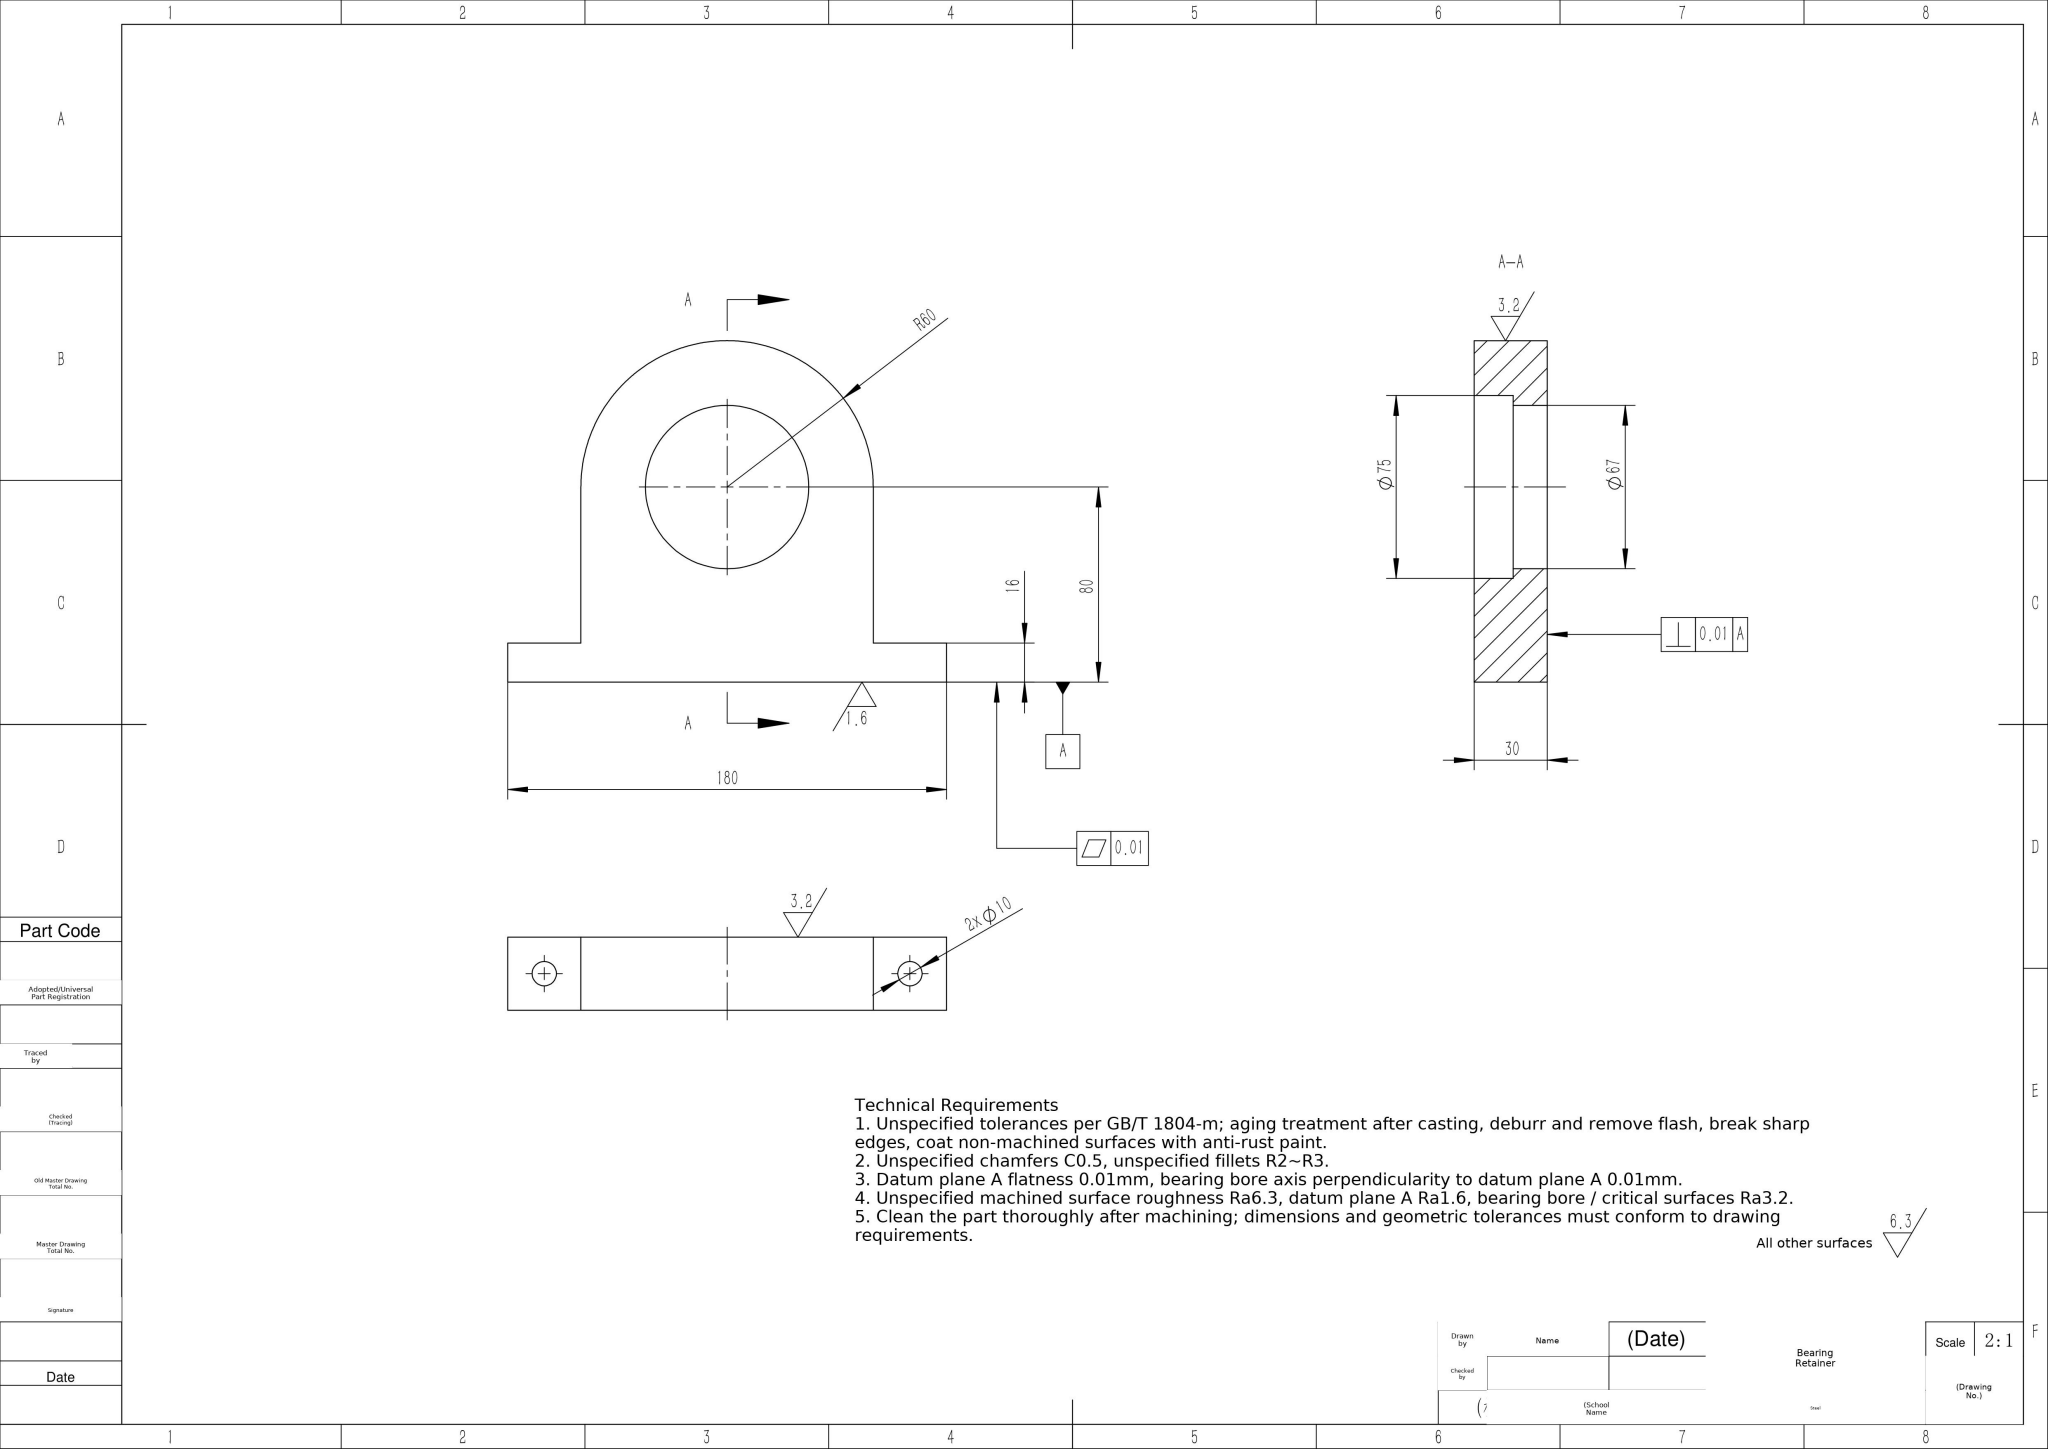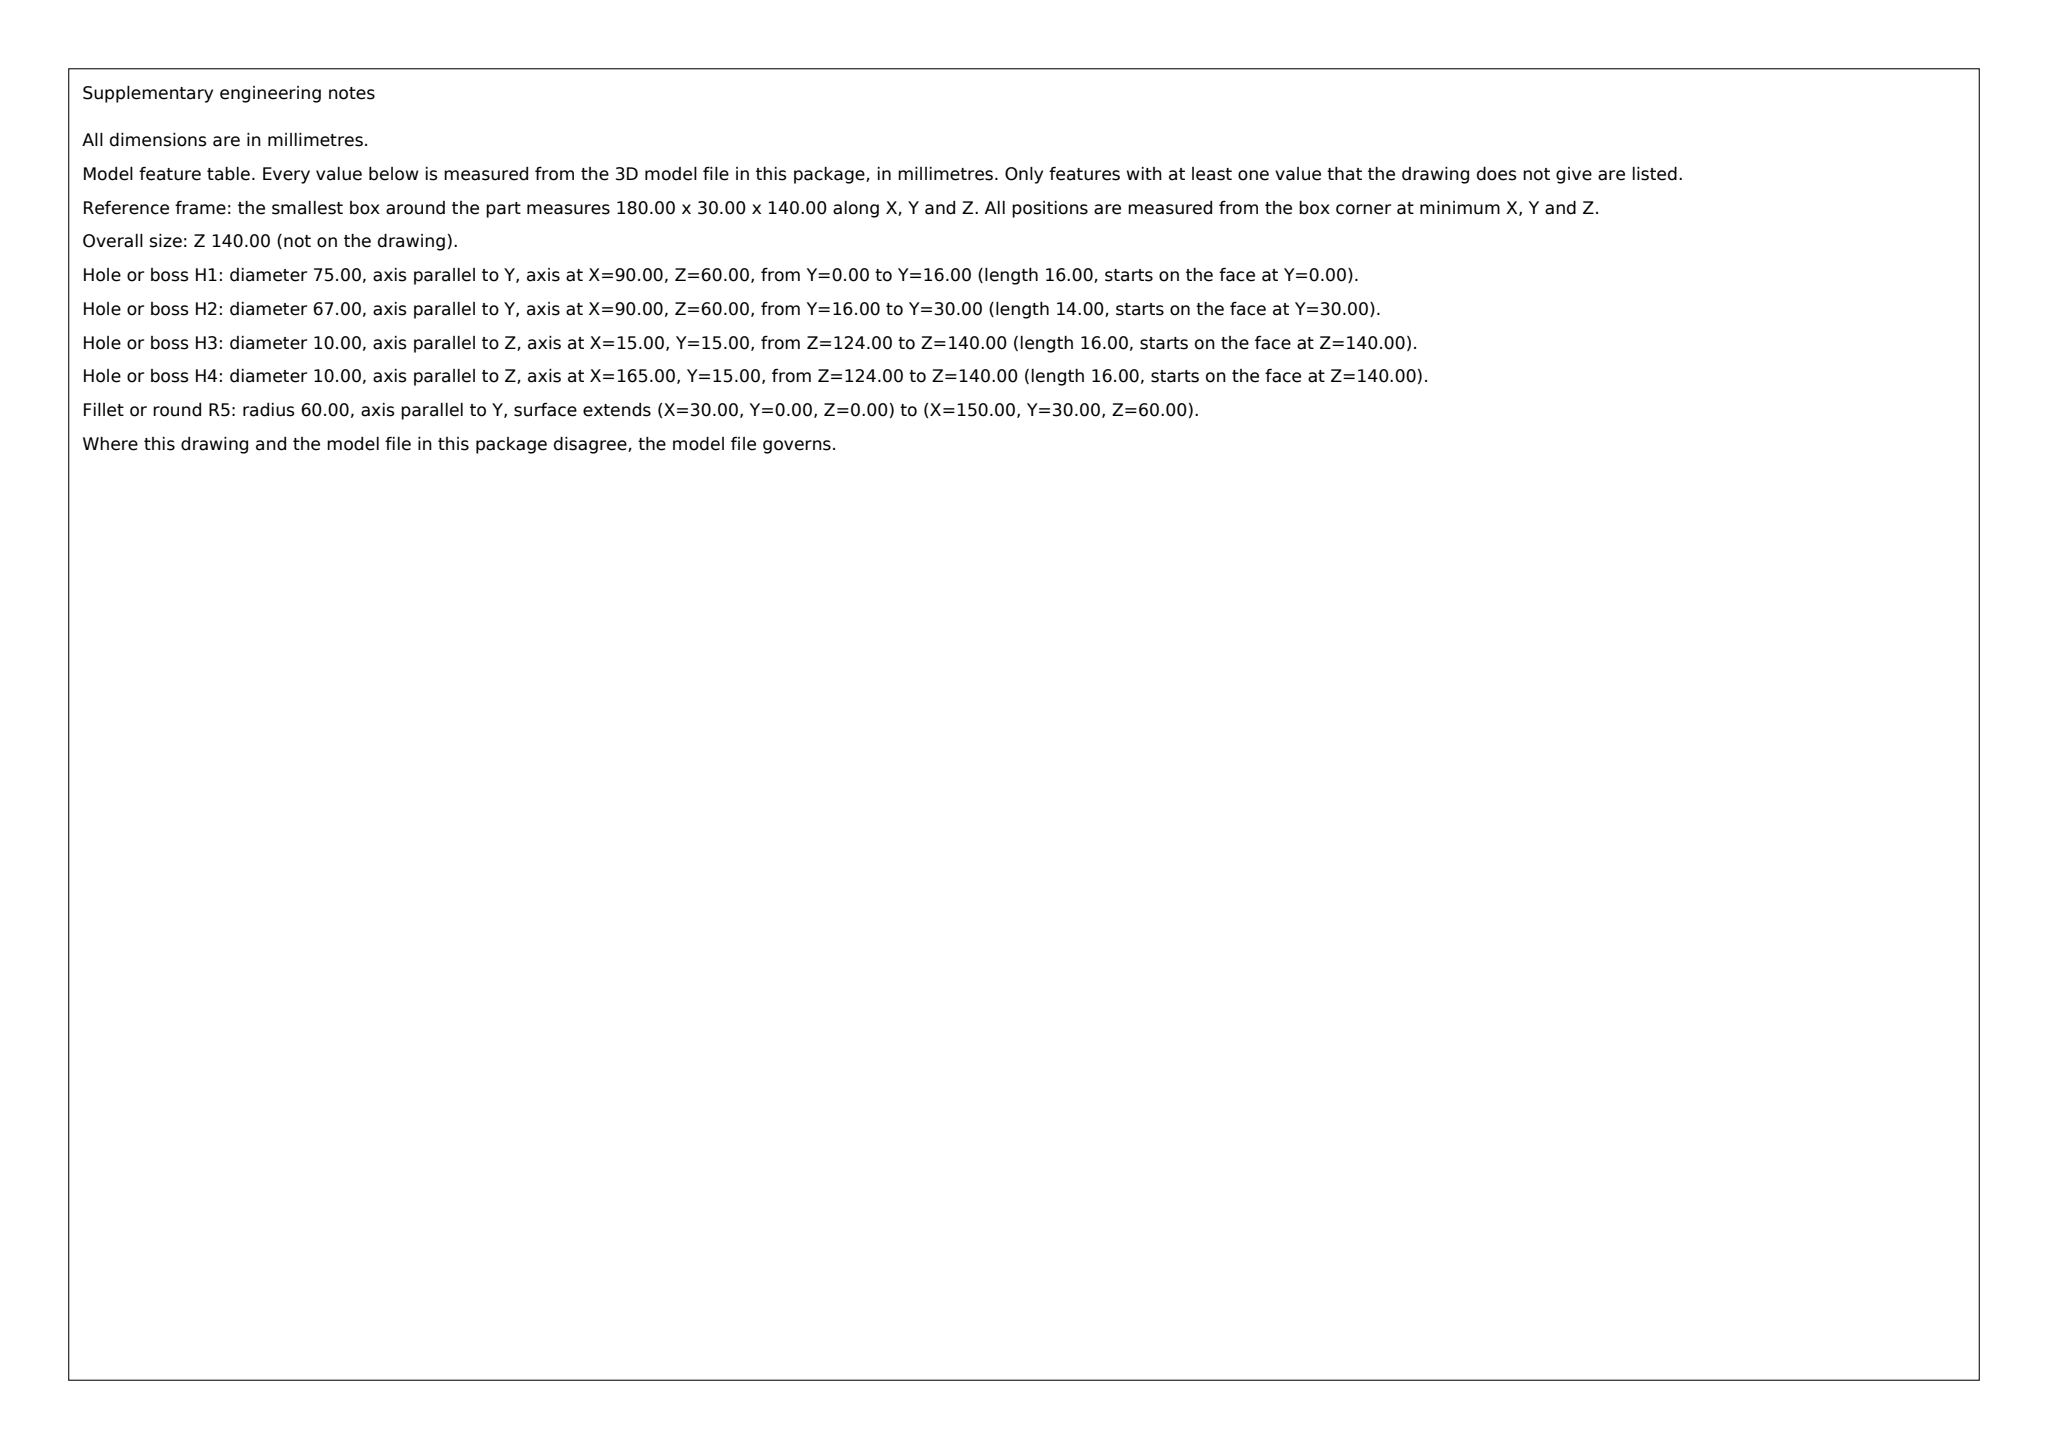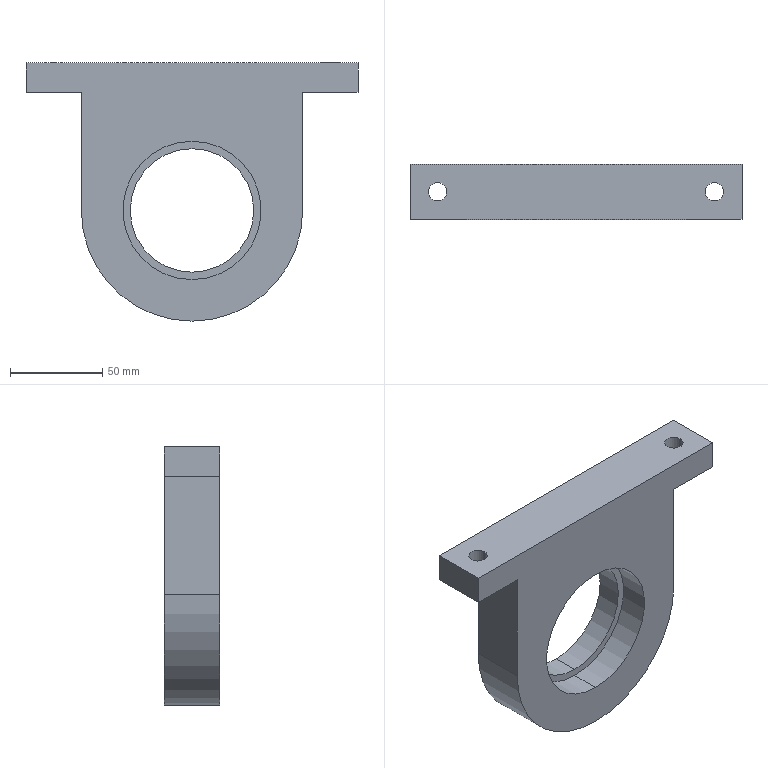Part | SolidWorks | mm | material Steel | 1 solid | 20 faces | box 180 x 30 x 140 mm | volume 363888 mm3 | cylinder 10 | plane 10 | commonest cylinder face diameters 10 x4 67 x2 120 x2 75 x2
build123d program:
from build123d import *

# Parameters (mm, degrees)
SKETCH1_R               = 37.5
BOSS_EXTRUDE1_DEPTH     = 30
BOSS_EXTRUDE2_START     = -14
SKETCH2_R               = 37.5
SKETCH2_R_2             = 33.5
BOSS_EXTRUDE2_DEPTH     = 14
SKETCH3_W               = 180
SKETCH3_H               = 30
BOSS_EXTRUDE3_DEPTH     = 16
CUT_EXTRUDE1_DEPTH      = 197.916
CUT_EXTRUDE1_DEPTH_BACK = 197.916
SKETCH4_R               = 5


with BuildPart() as part:
    # Sketch1 → Boss-Extrude1 (new body)
    with BuildSketch(Plane(origin=(0, 0, 0), x_dir=(1, 0, 0), z_dir=(0, 1, 0))):
        with BuildLine():
            Line((0, 0), (120, 0))
            Line((120, 0), (120, 80))
            ThreePointArc((120, 80), (60, 140), (0, 80))
            Line((0, 80), (0, 0))
        make_face()
        with Locations(Location((60, 80, 0), (0, 0, 270))):
            Circle(SKETCH1_R, mode=Mode.SUBTRACT)
    extrude(amount=BOSS_EXTRUDE1_DEPTH)

    # Sketch2 → Boss-Extrude2 (add)
    with BuildSketch(Plane(origin=(0, 30, 0), x_dir=(1, 0, 0), z_dir=(0, 1, 0)).offset(BOSS_EXTRUDE2_START)):
        with Locations(Location((60, 80, 0), (0, 0, 270))):
            Circle(SKETCH2_R)
        with Locations(Location((60, 80, 0), (0, 0, 270))):
            Circle(SKETCH2_R_2, mode=Mode.SUBTRACT)
    extrude(amount=BOSS_EXTRUDE2_DEPTH)

    # Sketch3 → Boss-Extrude3 (add)
    with BuildSketch(Plane.XY):
        with Locations((60, 15)):
            Rectangle(SKETCH3_W, SKETCH3_H)
    extrude(amount=-BOSS_EXTRUDE3_DEPTH)

    # Sketch4 → Cut-Extrude1 (cut, two sides: drawn at the far end of the back side and taken through both)
    with BuildSketch(Plane(origin=(0, 0, -16), x_dir=(-1, 0, 0), z_dir=(0, 0, -1)).offset(-CUT_EXTRUDE1_DEPTH_BACK)):
        with Locations((-135, 15)):
            Circle(SKETCH4_R)
        with Locations((15, 15)):
            Circle(SKETCH4_R)
    extrude(amount=CUT_EXTRUDE1_DEPTH + CUT_EXTRUDE1_DEPTH_BACK, mode=Mode.SUBTRACT)


solid = part.part
STEP:
#1=CARTESIAN_POINT('',(140.,15.,0.));
#2=VERTEX_POINT('',#1);
#3=CARTESIAN_POINT('',(130.,15.,0.));
#4=VERTEX_POINT('',#3);
#5=CARTESIAN_POINT('',(135.,15.,0.));
#6=DIRECTION('',(0.,0.,-1.));
#7=DIRECTION('',(-1.,0.,0.));
#8=AXIS2_PLACEMENT_3D('',#5,#6,#7);
#9=CIRCLE('',#8,5.);
#10=EDGE_CURVE('',#2,#4,#9,.T.);
#11=ORIENTED_EDGE('',*,*,#10,.F.);
#12=CARTESIAN_POINT('',(140.,15.,-16.));
#13=VERTEX_POINT('',#12);
#14=CARTESIAN_POINT('',(140.,15.,0.));
#15=DIRECTION('',(0.,0.,-1.));
#16=VECTOR('',#15,1000.);
#17=LINE('',#14,#16);
#18=EDGE_CURVE('',#2,#13,#17,.T.);
#19=ORIENTED_EDGE('',*,*,#18,.T.);
#20=CARTESIAN_POINT('',(130.,15.,-16.));
#21=VERTEX_POINT('',#20);
#22=CARTESIAN_POINT('',(135.,15.,-16.));
#23=DIRECTION('',(0.,0.,-1.));
#24=DIRECTION('',(-1.,0.,0.));
#25=AXIS2_PLACEMENT_3D('',#22,#23,#24);
#26=CIRCLE('',#25,5.);
#27=EDGE_CURVE('',#13,#21,#26,.T.);
#28=ORIENTED_EDGE('',*,*,#27,.T.);
#29=CARTESIAN_POINT('',(130.,15.,0.));
#30=DIRECTION('',(0.,0.,-1.));
#31=VECTOR('',#30,1000.);
#32=LINE('',#29,#31);
#33=EDGE_CURVE('',#4,#21,#32,.T.);
#34=ORIENTED_EDGE('',*,*,#33,.F.);
#35=EDGE_LOOP('',(#11,#19,#28,#34));
#36=FACE_OUTER_BOUND('',#35,.T.);
#37=CARTESIAN_POINT('',(135.,15.,0.));
#38=DIRECTION('',(0.,0.,-1.));
#39=DIRECTION('',(-1.,0.,0.));
#40=AXIS2_PLACEMENT_3D('',#37,#38,#39);
#41=CYLINDRICAL_SURFACE('',#40,5.);
#42=ADVANCED_FACE('',(#36),#41,.F.);
#43=CARTESIAN_POINT('',(-10.,15.,0.));
#44=VERTEX_POINT('',#43);
#45=CARTESIAN_POINT('',(-20.,15.,0.));
#46=VERTEX_POINT('',#45);
#47=CARTESIAN_POINT('',(-15.,15.,0.));
#48=DIRECTION('',(0.,0.,-1.));
#49=DIRECTION('',(-1.,0.,0.));
#50=AXIS2_PLACEMENT_3D('',#47,#48,#49);
#51=CIRCLE('',#50,5.);
#52=EDGE_CURVE('',#44,#46,#51,.T.);
#53=ORIENTED_EDGE('',*,*,#52,.F.);
#54=CARTESIAN_POINT('',(-10.,15.,-16.));
#55=VERTEX_POINT('',#54);
#56=CARTESIAN_POINT('',(-10.,15.,0.));
#57=DIRECTION('',(0.,0.,-1.));
#58=VECTOR('',#57,1000.);
#59=LINE('',#56,#58);
#60=EDGE_CURVE('',#44,#55,#59,.T.);
#61=ORIENTED_EDGE('',*,*,#60,.T.);
#62=CARTESIAN_POINT('',(-20.,15.,-16.));
#63=VERTEX_POINT('',#62);
#64=CARTESIAN_POINT('',(-15.,15.,-16.));
#65=DIRECTION('',(0.,0.,-1.));
#66=DIRECTION('',(-1.,0.,0.));
#67=AXIS2_PLACEMENT_3D('',#64,#65,#66);
#68=CIRCLE('',#67,5.);
#69=EDGE_CURVE('',#55,#63,#68,.T.);
#70=ORIENTED_EDGE('',*,*,#69,.T.);
#71=CARTESIAN_POINT('',(-20.,15.,0.));
#72=DIRECTION('',(0.,0.,-1.));
#73=VECTOR('',#72,1000.);
#74=LINE('',#71,#73);
#75=EDGE_CURVE('',#46,#63,#74,.T.);
#76=ORIENTED_EDGE('',*,*,#75,.F.);
#77=EDGE_LOOP('',(#53,#61,#70,#76));
#78=FACE_OUTER_BOUND('',#77,.T.);
#79=CARTESIAN_POINT('',(-15.,15.,0.));
#80=DIRECTION('',(0.,0.,-1.));
#81=DIRECTION('',(-1.,0.,0.));
#82=AXIS2_PLACEMENT_3D('',#79,#80,#81);
#83=CYLINDRICAL_SURFACE('',#82,5.);
#84=ADVANCED_FACE('',(#78),#83,.F.);
#85=CARTESIAN_POINT('',(60.,16.,-46.5));
#86=VERTEX_POINT('',#85);
#87=CARTESIAN_POINT('',(60.,16.,-113.5));
#88=VERTEX_POINT('',#87);
#89=CARTESIAN_POINT('',(60.,16.,-80.));
#90=DIRECTION('',(0.,-1.,0.));
#91=DIRECTION('',(0.,0.,1.));
#92=AXIS2_PLACEMENT_3D('',#89,#90,#91);
#93=CIRCLE('',#92,33.5);
#94=EDGE_CURVE('',#86,#88,#93,.T.);
#95=ORIENTED_EDGE('',*,*,#94,.T.);
#96=CARTESIAN_POINT('',(60.,30.,-113.5));
#97=VERTEX_POINT('',#96);
#98=CARTESIAN_POINT('',(60.,-106.066,-113.5));
#99=DIRECTION('',(0.,1.,0.));
#100=VECTOR('',#99,1000.);
#101=LINE('',#98,#100);
#102=EDGE_CURVE('',#88,#97,#101,.T.);
#103=ORIENTED_EDGE('',*,*,#102,.T.);
#104=CARTESIAN_POINT('',(60.,30.,-46.5));
#105=VERTEX_POINT('',#104);
#106=CARTESIAN_POINT('',(60.,30.,-80.));
#107=DIRECTION('',(0.,1.,0.));
#108=DIRECTION('',(0.,0.,1.));
#109=AXIS2_PLACEMENT_3D('',#106,#107,#108);
#110=CIRCLE('',#109,33.5);
#111=EDGE_CURVE('',#97,#105,#110,.T.);
#112=ORIENTED_EDGE('',*,*,#111,.T.);
#113=CARTESIAN_POINT('',(60.,-106.066,-46.5));
#114=DIRECTION('',(0.,1.,0.));
#115=VECTOR('',#114,1000.);
#116=LINE('',#113,#115);
#117=EDGE_CURVE('',#86,#105,#116,.T.);
#118=ORIENTED_EDGE('',*,*,#117,.F.);
#119=EDGE_LOOP('',(#95,#103,#112,#118));
#120=FACE_OUTER_BOUND('',#119,.T.);
#121=CARTESIAN_POINT('',(60.,-106.066,-80.));
#122=DIRECTION('',(0.,1.,0.));
#123=DIRECTION('',(0.,0.,1.));
#124=AXIS2_PLACEMENT_3D('',#121,#122,#123);
#125=CYLINDRICAL_SURFACE('',#124,33.5);
#126=ADVANCED_FACE('',(#120),#125,.F.);
#127=CARTESIAN_POINT('',(60.,30.,-140.));
#128=VERTEX_POINT('',#127);
#129=CARTESIAN_POINT('',(0.,30.,-80.));
#130=VERTEX_POINT('',#129);
#131=CARTESIAN_POINT('',(60.,30.,-80.));
#132=DIRECTION('',(0.,1.,0.));
#133=DIRECTION('',(0.,0.,1.));
#134=AXIS2_PLACEMENT_3D('',#131,#132,#133);
#135=CIRCLE('',#134,60.);
#136=EDGE_CURVE('',#128,#130,#135,.T.);
#137=ORIENTED_EDGE('',*,*,#136,.F.);
#138=CARTESIAN_POINT('',(60.,0.,-140.));
#139=VERTEX_POINT('',#138);
#140=CARTESIAN_POINT('',(60.,30.,-140.));
#141=DIRECTION('',(0.,-1.,0.));
#142=VECTOR('',#141,1000.);
#143=LINE('',#140,#142);
#144=EDGE_CURVE('',#128,#139,#143,.T.);
#145=ORIENTED_EDGE('',*,*,#144,.T.);
#146=CARTESIAN_POINT('',(0.,0.,-80.));
#147=VERTEX_POINT('',#146);
#148=CARTESIAN_POINT('',(60.,0.,-80.));
#149=DIRECTION('',(0.,1.,0.));
#150=DIRECTION('',(0.,0.,1.));
#151=AXIS2_PLACEMENT_3D('',#148,#149,#150);
#152=CIRCLE('',#151,60.);
#153=EDGE_CURVE('',#139,#147,#152,.T.);
#154=ORIENTED_EDGE('',*,*,#153,.T.);
#155=CARTESIAN_POINT('',(0.,30.,-80.));
#156=DIRECTION('',(0.,-1.,0.));
#157=VECTOR('',#156,1000.);
#158=LINE('',#155,#157);
#159=EDGE_CURVE('',#130,#147,#158,.T.);
#160=ORIENTED_EDGE('',*,*,#159,.F.);
#161=EDGE_LOOP('',(#137,#145,#154,#160));
#162=FACE_OUTER_BOUND('',#161,.T.);
#163=CARTESIAN_POINT('',(60.,30.,-80.));
#164=DIRECTION('',(0.,-1.,0.));
#165=DIRECTION('',(0.,0.,-1.));
#166=AXIS2_PLACEMENT_3D('',#163,#164,#165);
#167=CYLINDRICAL_SURFACE('',#166,60.);
#168=ADVANCED_FACE('',(#162),#167,.T.);
#169=CARTESIAN_POINT('',(60.,16.,-42.5));
#170=VERTEX_POINT('',#169);
#171=CARTESIAN_POINT('',(60.,16.,-117.5));
#172=VERTEX_POINT('',#171);
#173=CARTESIAN_POINT('',(60.,16.,-80.));
#174=DIRECTION('',(0.,-1.,0.));
#175=DIRECTION('',(0.,0.,1.));
#176=AXIS2_PLACEMENT_3D('',#173,#174,#175);
#177=CIRCLE('',#176,37.5);
#178=EDGE_CURVE('',#170,#172,#177,.T.);
#179=ORIENTED_EDGE('',*,*,#178,.F.);
#180=CARTESIAN_POINT('',(60.,0.,-42.5));
#181=VERTEX_POINT('',#180);
#182=CARTESIAN_POINT('',(60.,30.,-42.5));
#183=DIRECTION('',(0.,-1.,0.));
#184=VECTOR('',#183,1000.);
#185=LINE('',#182,#184);
#186=EDGE_CURVE('',#170,#181,#185,.T.);
#187=ORIENTED_EDGE('',*,*,#186,.T.);
#188=CARTESIAN_POINT('',(60.,0.,-117.5));
#189=VERTEX_POINT('',#188);
#190=CARTESIAN_POINT('',(60.,0.,-80.));
#191=DIRECTION('',(0.,1.,0.));
#192=DIRECTION('',(0.,0.,1.));
#193=AXIS2_PLACEMENT_3D('',#190,#191,#192);
#194=CIRCLE('',#193,37.5);
#195=EDGE_CURVE('',#189,#181,#194,.T.);
#196=ORIENTED_EDGE('',*,*,#195,.F.);
#197=CARTESIAN_POINT('',(60.,30.,-117.5));
#198=DIRECTION('',(0.,-1.,0.));
#199=VECTOR('',#198,1000.);
#200=LINE('',#197,#199);
#201=EDGE_CURVE('',#172,#189,#200,.T.);
#202=ORIENTED_EDGE('',*,*,#201,.F.);
#203=EDGE_LOOP('',(#179,#187,#196,#202));
#204=FACE_OUTER_BOUND('',#203,.T.);
#205=CARTESIAN_POINT('',(60.,30.,-80.));
#206=DIRECTION('',(0.,-1.,0.));
#207=DIRECTION('',(0.,0.,-1.));
#208=AXIS2_PLACEMENT_3D('',#205,#206,#207);
#209=CYLINDRICAL_SURFACE('',#208,37.5);
#210=ADVANCED_FACE('',(#204),#209,.F.);
#211=ORIENTED_EDGE('',*,*,#186,.F.);
#212=CARTESIAN_POINT('',(60.,16.,-80.));
#213=DIRECTION('',(0.,-1.,0.));
#214=DIRECTION('',(0.,0.,1.));
#215=AXIS2_PLACEMENT_3D('',#212,#213,#214);
#216=CIRCLE('',#215,37.5);
#217=EDGE_CURVE('',#172,#170,#216,.T.);
#218=ORIENTED_EDGE('',*,*,#217,.F.);
#219=ORIENTED_EDGE('',*,*,#201,.T.);
#220=CARTESIAN_POINT('',(60.,0.,-80.));
#221=DIRECTION('',(0.,1.,0.));
#222=DIRECTION('',(0.,0.,1.));
#223=AXIS2_PLACEMENT_3D('',#220,#221,#222);
#224=CIRCLE('',#223,37.5);
#225=EDGE_CURVE('',#181,#189,#224,.T.);
#226=ORIENTED_EDGE('',*,*,#225,.F.);
#227=EDGE_LOOP('',(#211,#218,#219,#226));
#228=FACE_OUTER_BOUND('',#227,.T.);
#229=CARTESIAN_POINT('',(60.,30.,-80.));
#230=DIRECTION('',(0.,-1.,0.));
#231=DIRECTION('',(0.,0.,-1.));
#232=AXIS2_PLACEMENT_3D('',#229,#230,#231);
#233=CYLINDRICAL_SURFACE('',#232,37.5);
#234=ADVANCED_FACE('',(#228),#233,.F.);
#235=CARTESIAN_POINT('',(-0.,30.,-16.));
#236=VERTEX_POINT('',#235);
#237=CARTESIAN_POINT('',(0.,30.,0.));
#238=DIRECTION('',(0.,0.,1.));
#239=VECTOR('',#238,1000.);
#240=LINE('',#237,#239);
#241=EDGE_CURVE('',#130,#236,#240,.T.);
#242=ORIENTED_EDGE('',*,*,#241,.T.);
#243=CARTESIAN_POINT('',(-30.,30.,-16.));
#244=VERTEX_POINT('',#243);
#245=CARTESIAN_POINT('',(-30.,30.,-16.));
#246=DIRECTION('',(-1.,0.,0.));
#247=VECTOR('',#246,1000.);
#248=LINE('',#245,#247);
#249=EDGE_CURVE('',#236,#244,#248,.T.);
#250=ORIENTED_EDGE('',*,*,#249,.T.);
#251=CARTESIAN_POINT('',(-30.,30.,0.));
#252=VERTEX_POINT('',#251);
#253=CARTESIAN_POINT('',(-30.,30.,-16.));
#254=DIRECTION('',(0.,0.,1.));
#255=VECTOR('',#254,1000.);
#256=LINE('',#253,#255);
#257=EDGE_CURVE('',#244,#252,#256,.T.);
#258=ORIENTED_EDGE('',*,*,#257,.T.);
#259=CARTESIAN_POINT('',(150.,30.,0.));
#260=VERTEX_POINT('',#259);
#261=CARTESIAN_POINT('',(0.,30.,0.));
#262=DIRECTION('',(1.,0.,0.));
#263=VECTOR('',#262,1000.);
#264=LINE('',#261,#263);
#265=EDGE_CURVE('',#252,#260,#264,.T.);
#266=ORIENTED_EDGE('',*,*,#265,.T.);
#267=CARTESIAN_POINT('',(150.,30.,-16.));
#268=VERTEX_POINT('',#267);
#269=CARTESIAN_POINT('',(150.,30.,-16.));
#270=DIRECTION('',(0.,0.,1.));
#271=VECTOR('',#270,1000.);
#272=LINE('',#269,#271);
#273=EDGE_CURVE('',#268,#260,#272,.T.);
#274=ORIENTED_EDGE('',*,*,#273,.F.);
#275=CARTESIAN_POINT('',(120.,30.,-16.));
#276=VERTEX_POINT('',#275);
#277=CARTESIAN_POINT('',(-30.,30.,-16.));
#278=DIRECTION('',(-1.,0.,0.));
#279=VECTOR('',#278,1000.);
#280=LINE('',#277,#279);
#281=EDGE_CURVE('',#268,#276,#280,.T.);
#282=ORIENTED_EDGE('',*,*,#281,.T.);
#283=CARTESIAN_POINT('',(120.,30.,-80.));
#284=VERTEX_POINT('',#283);
#285=CARTESIAN_POINT('',(120.,30.,0.));
#286=DIRECTION('',(0.,0.,-1.));
#287=VECTOR('',#286,1000.);
#288=LINE('',#285,#287);
#289=EDGE_CURVE('',#276,#284,#288,.T.);
#290=ORIENTED_EDGE('',*,*,#289,.T.);
#291=CARTESIAN_POINT('',(60.,30.,-80.));
#292=DIRECTION('',(0.,1.,0.));
#293=DIRECTION('',(0.,0.,1.));
#294=AXIS2_PLACEMENT_3D('',#291,#292,#293);
#295=CIRCLE('',#294,60.);
#296=EDGE_CURVE('',#284,#128,#295,.T.);
#297=ORIENTED_EDGE('',*,*,#296,.T.);
#298=ORIENTED_EDGE('',*,*,#136,.T.);
#299=EDGE_LOOP('',(#242,#250,#258,#266,#274,#282,#290,#297,#298));
#300=FACE_OUTER_BOUND('',#299,.T.);
#301=CARTESIAN_POINT('',(60.,30.,-80.));
#302=DIRECTION('',(0.,1.,0.));
#303=DIRECTION('',(0.,0.,1.));
#304=AXIS2_PLACEMENT_3D('',#301,#302,#303);
#305=CIRCLE('',#304,33.5);
#306=EDGE_CURVE('',#105,#97,#305,.T.);
#307=ORIENTED_EDGE('',*,*,#306,.F.);
#308=ORIENTED_EDGE('',*,*,#111,.F.);
#309=EDGE_LOOP('',(#307,#308));
#310=FACE_BOUND('',#309,.T.);
#311=CARTESIAN_POINT('',(60.,30.,-80.));
#312=DIRECTION('',(0.,1.,0.));
#313=DIRECTION('',(0.,0.,1.));
#314=AXIS2_PLACEMENT_3D('',#311,#312,#313);
#315=PLANE('',#314);
#316=ADVANCED_FACE('',(#300,#310),#315,.T.);
#317=CARTESIAN_POINT('',(120.,0.,-16.));
#318=VERTEX_POINT('',#317);
#319=CARTESIAN_POINT('',(120.,0.,-80.));
#320=VERTEX_POINT('',#319);
#321=CARTESIAN_POINT('',(120.,0.,0.));
#322=DIRECTION('',(0.,0.,-1.));
#323=VECTOR('',#322,1000.);
#324=LINE('',#321,#323);
#325=EDGE_CURVE('',#318,#320,#324,.T.);
#326=ORIENTED_EDGE('',*,*,#325,.F.);
#327=CARTESIAN_POINT('',(150.,0.,-16.));
#328=VERTEX_POINT('',#327);
#329=CARTESIAN_POINT('',(-30.,0.,-16.));
#330=DIRECTION('',(1.,0.,0.));
#331=VECTOR('',#330,1000.);
#332=LINE('',#329,#331);
#333=EDGE_CURVE('',#318,#328,#332,.T.);
#334=ORIENTED_EDGE('',*,*,#333,.T.);
#335=CARTESIAN_POINT('',(150.,0.,0.));
#336=VERTEX_POINT('',#335);
#337=CARTESIAN_POINT('',(150.,0.,-16.));
#338=DIRECTION('',(0.,0.,1.));
#339=VECTOR('',#338,1000.);
#340=LINE('',#337,#339);
#341=EDGE_CURVE('',#328,#336,#340,.T.);
#342=ORIENTED_EDGE('',*,*,#341,.T.);
#343=CARTESIAN_POINT('',(-30.,0.,0.));
#344=VERTEX_POINT('',#343);
#345=CARTESIAN_POINT('',(0.,0.,0.));
#346=DIRECTION('',(1.,0.,0.));
#347=VECTOR('',#346,1000.);
#348=LINE('',#345,#347);
#349=EDGE_CURVE('',#344,#336,#348,.T.);
#350=ORIENTED_EDGE('',*,*,#349,.F.);
#351=CARTESIAN_POINT('',(-30.,0.,-16.));
#352=VERTEX_POINT('',#351);
#353=CARTESIAN_POINT('',(-30.,0.,-16.));
#354=DIRECTION('',(0.,0.,1.));
#355=VECTOR('',#354,1000.);
#356=LINE('',#353,#355);
#357=EDGE_CURVE('',#352,#344,#356,.T.);
#358=ORIENTED_EDGE('',*,*,#357,.F.);
#359=CARTESIAN_POINT('',(-0.,0.,-16.));
#360=VERTEX_POINT('',#359);
#361=CARTESIAN_POINT('',(-30.,0.,-16.));
#362=DIRECTION('',(1.,0.,0.));
#363=VECTOR('',#362,1000.);
#364=LINE('',#361,#363);
#365=EDGE_CURVE('',#352,#360,#364,.T.);
#366=ORIENTED_EDGE('',*,*,#365,.T.);
#367=CARTESIAN_POINT('',(0.,0.,0.));
#368=DIRECTION('',(0.,0.,1.));
#369=VECTOR('',#368,1000.);
#370=LINE('',#367,#369);
#371=EDGE_CURVE('',#147,#360,#370,.T.);
#372=ORIENTED_EDGE('',*,*,#371,.F.);
#373=ORIENTED_EDGE('',*,*,#153,.F.);
#374=CARTESIAN_POINT('',(60.,0.,-80.));
#375=DIRECTION('',(0.,1.,0.));
#376=DIRECTION('',(0.,0.,1.));
#377=AXIS2_PLACEMENT_3D('',#374,#375,#376);
#378=CIRCLE('',#377,60.);
#379=EDGE_CURVE('',#320,#139,#378,.T.);
#380=ORIENTED_EDGE('',*,*,#379,.F.);
#381=EDGE_LOOP('',(#326,#334,#342,#350,#358,#366,#372,#373,#380));
#382=FACE_OUTER_BOUND('',#381,.T.);
#383=ORIENTED_EDGE('',*,*,#195,.T.);
#384=ORIENTED_EDGE('',*,*,#225,.T.);
#385=EDGE_LOOP('',(#383,#384));
#386=FACE_BOUND('',#385,.T.);
#387=CARTESIAN_POINT('',(60.,0.,-80.));
#388=DIRECTION('',(0.,1.,0.));
#389=DIRECTION('',(0.,0.,1.));
#390=AXIS2_PLACEMENT_3D('',#387,#388,#389);
#391=PLANE('',#390);
#392=ADVANCED_FACE('',(#382,#386),#391,.F.);
#393=ORIENTED_EDGE('',*,*,#371,.T.);
#394=CARTESIAN_POINT('',(0.,30.,-16.));
#395=DIRECTION('',(0.,1.,0.));
#396=VECTOR('',#395,1000.);
#397=LINE('',#394,#396);
#398=EDGE_CURVE('',#360,#236,#397,.T.);
#399=ORIENTED_EDGE('',*,*,#398,.T.);
#400=ORIENTED_EDGE('',*,*,#241,.F.);
#401=ORIENTED_EDGE('',*,*,#159,.T.);
#402=EDGE_LOOP('',(#393,#399,#400,#401));
#403=FACE_OUTER_BOUND('',#402,.T.);
#404=CARTESIAN_POINT('',(0.,30.,0.));
#405=DIRECTION('',(1.,0.,0.));
#406=DIRECTION('',(0.,0.,-1.));
#407=AXIS2_PLACEMENT_3D('',#404,#405,#406);
#408=PLANE('',#407);
#409=ADVANCED_FACE('',(#403),#408,.F.);
#410=CARTESIAN_POINT('',(135.,15.,0.));
#411=DIRECTION('',(0.,0.,-1.));
#412=DIRECTION('',(-1.,0.,0.));
#413=AXIS2_PLACEMENT_3D('',#410,#411,#412);
#414=CIRCLE('',#413,5.);
#415=EDGE_CURVE('',#4,#2,#414,.T.);
#416=ORIENTED_EDGE('',*,*,#415,.T.);
#417=ORIENTED_EDGE('',*,*,#10,.T.);
#418=EDGE_LOOP('',(#416,#417));
#419=FACE_BOUND('',#418,.T.);
#420=CARTESIAN_POINT('',(-15.,15.,0.));
#421=DIRECTION('',(0.,0.,-1.));
#422=DIRECTION('',(-1.,0.,0.));
#423=AXIS2_PLACEMENT_3D('',#420,#421,#422);
#424=CIRCLE('',#423,5.);
#425=EDGE_CURVE('',#46,#44,#424,.T.);
#426=ORIENTED_EDGE('',*,*,#425,.T.);
#427=ORIENTED_EDGE('',*,*,#52,.T.);
#428=EDGE_LOOP('',(#426,#427));
#429=FACE_BOUND('',#428,.T.);
#430=ORIENTED_EDGE('',*,*,#349,.T.);
#431=CARTESIAN_POINT('',(150.,0.,0.));
#432=DIRECTION('',(0.,1.,0.));
#433=VECTOR('',#432,1000.);
#434=LINE('',#431,#433);
#435=EDGE_CURVE('',#336,#260,#434,.T.);
#436=ORIENTED_EDGE('',*,*,#435,.T.);
#437=ORIENTED_EDGE('',*,*,#265,.F.);
#438=CARTESIAN_POINT('',(-30.,0.,0.));
#439=DIRECTION('',(0.,-1.,0.));
#440=VECTOR('',#439,1000.);
#441=LINE('',#438,#440);
#442=EDGE_CURVE('',#252,#344,#441,.T.);
#443=ORIENTED_EDGE('',*,*,#442,.T.);
#444=EDGE_LOOP('',(#430,#436,#437,#443));
#445=FACE_OUTER_BOUND('',#444,.T.);
#446=CARTESIAN_POINT('',(0.,30.,0.));
#447=DIRECTION('',(0.,0.,-1.));
#448=DIRECTION('',(-1.,0.,0.));
#449=AXIS2_PLACEMENT_3D('',#446,#447,#448);
#450=PLANE('',#449);
#451=ADVANCED_FACE('',(#419,#429,#445),#450,.F.);
#452=ORIENTED_EDGE('',*,*,#289,.F.);
#453=CARTESIAN_POINT('',(120.,30.,-16.));
#454=DIRECTION('',(0.,-1.,0.));
#455=VECTOR('',#454,1000.);
#456=LINE('',#453,#455);
#457=EDGE_CURVE('',#276,#318,#456,.T.);
#458=ORIENTED_EDGE('',*,*,#457,.T.);
#459=ORIENTED_EDGE('',*,*,#325,.T.);
#460=CARTESIAN_POINT('',(120.,30.,-80.));
#461=DIRECTION('',(0.,-1.,0.));
#462=VECTOR('',#461,1000.);
#463=LINE('',#460,#462);
#464=EDGE_CURVE('',#284,#320,#463,.T.);
#465=ORIENTED_EDGE('',*,*,#464,.F.);
#466=EDGE_LOOP('',(#452,#458,#459,#465));
#467=FACE_OUTER_BOUND('',#466,.T.);
#468=CARTESIAN_POINT('',(120.,30.,0.));
#469=DIRECTION('',(-1.,0.,0.));
#470=DIRECTION('',(0.,0.,1.));
#471=AXIS2_PLACEMENT_3D('',#468,#469,#470);
#472=PLANE('',#471);
#473=ADVANCED_FACE('',(#467),#472,.F.);
#474=ORIENTED_EDGE('',*,*,#144,.F.);
#475=ORIENTED_EDGE('',*,*,#296,.F.);
#476=ORIENTED_EDGE('',*,*,#464,.T.);
#477=ORIENTED_EDGE('',*,*,#379,.T.);
#478=EDGE_LOOP('',(#474,#475,#476,#477));
#479=FACE_OUTER_BOUND('',#478,.T.);
#480=CARTESIAN_POINT('',(60.,30.,-80.));
#481=DIRECTION('',(0.,-1.,0.));
#482=DIRECTION('',(0.,0.,-1.));
#483=AXIS2_PLACEMENT_3D('',#480,#481,#482);
#484=CYLINDRICAL_SURFACE('',#483,60.);
#485=ADVANCED_FACE('',(#479),#484,.T.);
#486=ORIENTED_EDGE('',*,*,#102,.F.);
#487=CARTESIAN_POINT('',(60.,16.,-80.));
#488=DIRECTION('',(0.,-1.,0.));
#489=DIRECTION('',(0.,0.,1.));
#490=AXIS2_PLACEMENT_3D('',#487,#488,#489);
#491=CIRCLE('',#490,33.5);
#492=EDGE_CURVE('',#88,#86,#491,.T.);
#493=ORIENTED_EDGE('',*,*,#492,.T.);
#494=ORIENTED_EDGE('',*,*,#117,.T.);
#495=ORIENTED_EDGE('',*,*,#306,.T.);
#496=EDGE_LOOP('',(#486,#493,#494,#495));
#497=FACE_OUTER_BOUND('',#496,.T.);
#498=CARTESIAN_POINT('',(60.,-106.066,-80.));
#499=DIRECTION('',(0.,1.,0.));
#500=DIRECTION('',(0.,0.,1.));
#501=AXIS2_PLACEMENT_3D('',#498,#499,#500);
#502=CYLINDRICAL_SURFACE('',#501,33.5);
#503=ADVANCED_FACE('',(#497),#502,.F.);
#504=ORIENTED_EDGE('',*,*,#217,.T.);
#505=ORIENTED_EDGE('',*,*,#178,.T.);
#506=EDGE_LOOP('',(#504,#505));
#507=FACE_OUTER_BOUND('',#506,.T.);
#508=ORIENTED_EDGE('',*,*,#94,.F.);
#509=ORIENTED_EDGE('',*,*,#492,.F.);
#510=EDGE_LOOP('',(#508,#509));
#511=FACE_BOUND('',#510,.T.);
#512=CARTESIAN_POINT('',(60.,16.,-80.));
#513=DIRECTION('',(0.,1.,0.));
#514=DIRECTION('',(0.,0.,1.));
#515=AXIS2_PLACEMENT_3D('',#512,#513,#514);
#516=PLANE('',#515);
#517=ADVANCED_FACE('',(#507,#511),#516,.F.);
#518=ORIENTED_EDGE('',*,*,#435,.F.);
#519=ORIENTED_EDGE('',*,*,#341,.F.);
#520=CARTESIAN_POINT('',(150.,0.,-16.));
#521=DIRECTION('',(0.,1.,0.));
#522=VECTOR('',#521,1000.);
#523=LINE('',#520,#522);
#524=EDGE_CURVE('',#328,#268,#523,.T.);
#525=ORIENTED_EDGE('',*,*,#524,.T.);
#526=ORIENTED_EDGE('',*,*,#273,.T.);
#527=EDGE_LOOP('',(#518,#519,#525,#526));
#528=FACE_OUTER_BOUND('',#527,.T.);
#529=CARTESIAN_POINT('',(150.,0.,-16.));
#530=DIRECTION('',(1.,0.,0.));
#531=DIRECTION('',(0.,0.,-1.));
#532=AXIS2_PLACEMENT_3D('',#529,#530,#531);
#533=PLANE('',#532);
#534=ADVANCED_FACE('',(#528),#533,.T.);
#535=CARTESIAN_POINT('',(135.,15.,-16.));
#536=DIRECTION('',(0.,0.,-1.));
#537=DIRECTION('',(-1.,0.,0.));
#538=AXIS2_PLACEMENT_3D('',#535,#536,#537);
#539=CIRCLE('',#538,5.);
#540=EDGE_CURVE('',#21,#13,#539,.T.);
#541=ORIENTED_EDGE('',*,*,#540,.F.);
#542=ORIENTED_EDGE('',*,*,#27,.F.);
#543=EDGE_LOOP('',(#541,#542));
#544=FACE_BOUND('',#543,.T.);
#545=ORIENTED_EDGE('',*,*,#457,.F.);
#546=ORIENTED_EDGE('',*,*,#281,.F.);
#547=ORIENTED_EDGE('',*,*,#524,.F.);
#548=ORIENTED_EDGE('',*,*,#333,.F.);
#549=EDGE_LOOP('',(#545,#546,#547,#548));
#550=FACE_OUTER_BOUND('',#549,.T.);
#551=CARTESIAN_POINT('',(0.,0.,-16.));
#552=DIRECTION('',(0.,0.,-1.));
#553=DIRECTION('',(-1.,0.,0.));
#554=AXIS2_PLACEMENT_3D('',#551,#552,#553);
#555=PLANE('',#554);
#556=ADVANCED_FACE('',(#544,#550),#555,.T.);
#557=CARTESIAN_POINT('',(-15.,15.,-16.));
#558=DIRECTION('',(0.,0.,-1.));
#559=DIRECTION('',(-1.,0.,0.));
#560=AXIS2_PLACEMENT_3D('',#557,#558,#559);
#561=CIRCLE('',#560,5.);
#562=EDGE_CURVE('',#63,#55,#561,.T.);
#563=ORIENTED_EDGE('',*,*,#562,.F.);
#564=ORIENTED_EDGE('',*,*,#69,.F.);
#565=EDGE_LOOP('',(#563,#564));
#566=FACE_BOUND('',#565,.T.);
#567=ORIENTED_EDGE('',*,*,#398,.F.);
#568=ORIENTED_EDGE('',*,*,#365,.F.);
#569=CARTESIAN_POINT('',(-30.,0.,-16.));
#570=DIRECTION('',(0.,-1.,0.));
#571=VECTOR('',#570,1000.);
#572=LINE('',#569,#571);
#573=EDGE_CURVE('',#244,#352,#572,.T.);
#574=ORIENTED_EDGE('',*,*,#573,.F.);
#575=ORIENTED_EDGE('',*,*,#249,.F.);
#576=EDGE_LOOP('',(#567,#568,#574,#575));
#577=FACE_OUTER_BOUND('',#576,.T.);
#578=CARTESIAN_POINT('',(0.,0.,-16.));
#579=DIRECTION('',(0.,0.,-1.));
#580=DIRECTION('',(-1.,0.,0.));
#581=AXIS2_PLACEMENT_3D('',#578,#579,#580);
#582=PLANE('',#581);
#583=ADVANCED_FACE('',(#566,#577),#582,.T.);
#584=ORIENTED_EDGE('',*,*,#442,.F.);
#585=ORIENTED_EDGE('',*,*,#257,.F.);
#586=ORIENTED_EDGE('',*,*,#573,.T.);
#587=ORIENTED_EDGE('',*,*,#357,.T.);
#588=EDGE_LOOP('',(#584,#585,#586,#587));
#589=FACE_OUTER_BOUND('',#588,.T.);
#590=CARTESIAN_POINT('',(-30.,0.,-16.));
#591=DIRECTION('',(-1.,0.,0.));
#592=DIRECTION('',(0.,0.,1.));
#593=AXIS2_PLACEMENT_3D('',#590,#591,#592);
#594=PLANE('',#593);
#595=ADVANCED_FACE('',(#589),#594,.T.);
#596=ORIENTED_EDGE('',*,*,#60,.F.);
#597=ORIENTED_EDGE('',*,*,#425,.F.);
#598=ORIENTED_EDGE('',*,*,#75,.T.);
#599=ORIENTED_EDGE('',*,*,#562,.T.);
#600=EDGE_LOOP('',(#596,#597,#598,#599));
#601=FACE_OUTER_BOUND('',#600,.T.);
#602=CARTESIAN_POINT('',(-15.,15.,0.));
#603=DIRECTION('',(0.,0.,-1.));
#604=DIRECTION('',(-1.,0.,0.));
#605=AXIS2_PLACEMENT_3D('',#602,#603,#604);
#606=CYLINDRICAL_SURFACE('',#605,5.);
#607=ADVANCED_FACE('',(#601),#606,.F.);
#608=ORIENTED_EDGE('',*,*,#18,.F.);
#609=ORIENTED_EDGE('',*,*,#415,.F.);
#610=ORIENTED_EDGE('',*,*,#33,.T.);
#611=ORIENTED_EDGE('',*,*,#540,.T.);
#612=EDGE_LOOP('',(#608,#609,#610,#611));
#613=FACE_OUTER_BOUND('',#612,.T.);
#614=CARTESIAN_POINT('',(135.,15.,0.));
#615=DIRECTION('',(0.,0.,-1.));
#616=DIRECTION('',(-1.,0.,0.));
#617=AXIS2_PLACEMENT_3D('',#614,#615,#616);
#618=CYLINDRICAL_SURFACE('',#617,5.);
#619=ADVANCED_FACE('',(#613),#618,.F.);
#620=CLOSED_SHELL('',(#42,#84,#126,#168,#210,#234,#316,#392,#409,#451,#473,#485,#503,#517,#534,#556,#583,#595,#607,#619));
#621=MANIFOLD_SOLID_BREP('',#620);
#622=CARTESIAN_POINT('',(0.,0.,0.));
#623=DIRECTION('',(0.,0.,1.));
#624=DIRECTION('',(1.,0.,0.));
#625=AXIS2_PLACEMENT_3D('',#622,#623,#624);
#626=(LENGTH_UNIT()NAMED_UNIT(*)SI_UNIT(.MILLI.,.METRE.));
#627=UNCERTAINTY_MEASURE_WITH_UNIT(LENGTH_MEASURE(0.00001),#626,'','');
#628=(NAMED_UNIT(*)PLANE_ANGLE_UNIT()SI_UNIT($,.RADIAN.));
#629=(NAMED_UNIT(*)SI_UNIT($,.STERADIAN.)SOLID_ANGLE_UNIT());
#630=(GEOMETRIC_REPRESENTATION_CONTEXT(3)GLOBAL_UNCERTAINTY_ASSIGNED_CONTEXT((#627))GLOBAL_UNIT_ASSIGNED_CONTEXT((#626,#628,#629))REPRESENTATION_CONTEXT('',''));
#631=ADVANCED_BREP_SHAPE_REPRESENTATION('',(#621,#625),#630);